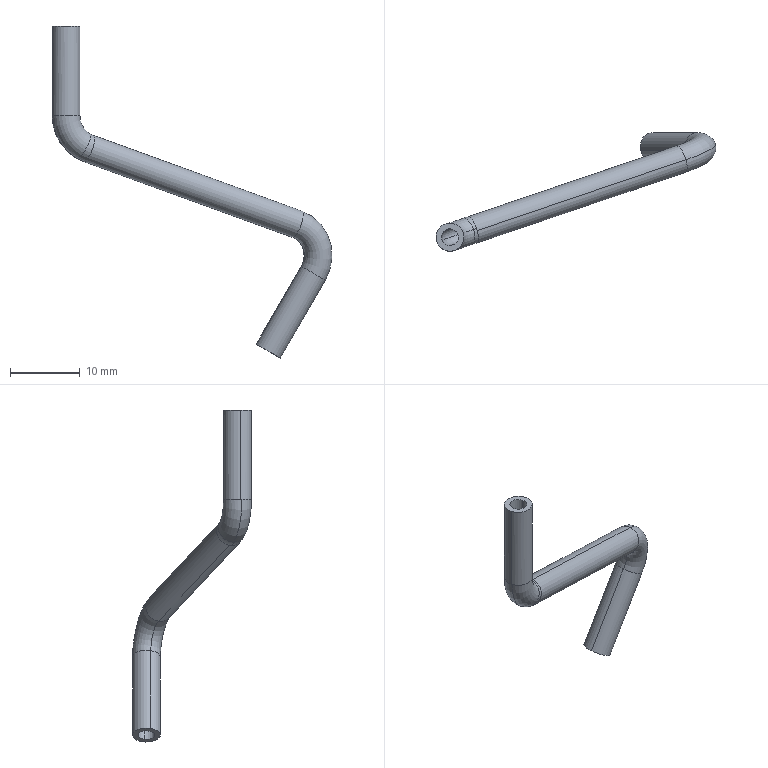Component | SolidWorks | WaterPipe6-1 | 1 solid | 26 faces | box 40.18 x 17.05 x 47.64 mm | volume 596 mm3 | torus 12 | cylinder 12 | plane 2 | commonest cylinder face diameters 2.4 x6 4 x6
build123d program:
from build123d import *

# Parameters (mm, degrees)
SCAN_THIN_FEATURE1_PROFILE_R   = 2
SCAN_THIN_FEATURE1_PROFILE_R_2 = 1.2


with BuildPart() as part:
    # Scan-Thin Feature1: sweep along a curve in space
    with BuildLine() as scan_thin_feature1_path:
        Line((0, 0, 0), (0, 0, -12.897))
        ThreePointArc((5.829, -0.1672, -17.827), (1.771, -0.05079, -16.715), (0, 0, -12.897))
        Line((5.829, -0.1672, -17.827), (38.795, -1.113, -12.268))
        ThreePointArc((44.025, -0.7122, -14.766), (41.815, -1.048, -12.69), (38.795, -1.113, -12.268))
        Line((44.025, -0.7122, -14.766), (50.182, 1.091, -25.878))
    # Scan-Thin Feature1 profile (on start of the path) → Scan-Thin Feature1 (sweep)
    with BuildSketch(Plane(origin=(0, 0, 0), x_dir=(-1, 0, 0), z_dir=(0, 0, -1))):
        Circle(SCAN_THIN_FEATURE1_PROFILE_R)
        Circle(SCAN_THIN_FEATURE1_PROFILE_R_2, mode=Mode.SUBTRACT)
    sweep(path=scan_thin_feature1_path.line)


solid = part.part

# Placed as in the assembly
solid = solid.moved(Location((23.053, 33.561, 100.756), (180, -30, 163.68)))